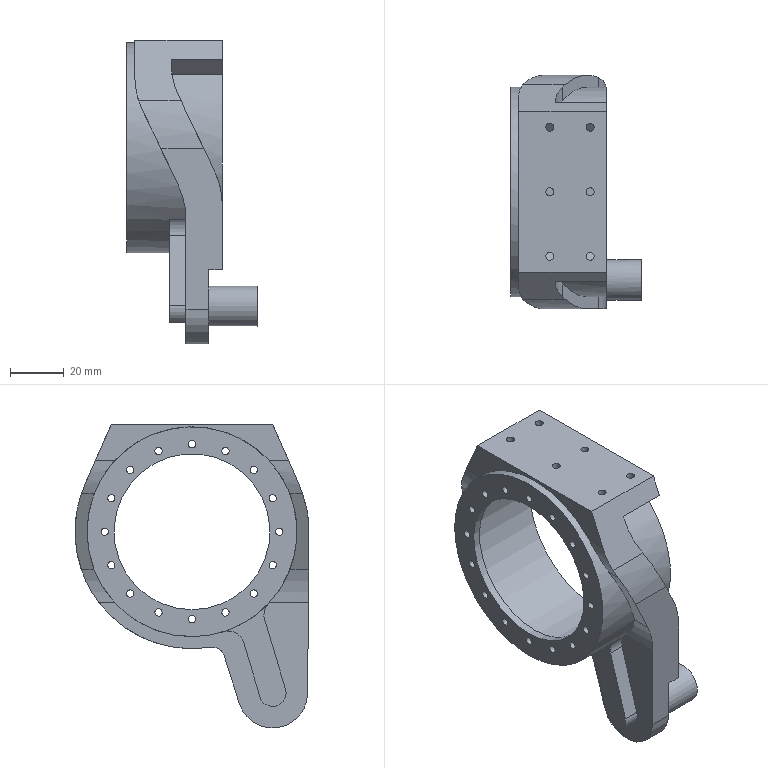Component | NX | TILT_BASE_ACC_1 | 1 solid | 74 faces | volume 76089 mm3 | cylinder 45 | plane 29 | commonest cylinder face diameters 2.7 x16 57 x8 3 x6 78 x3 87 x2 12 x2 70 x1 9 x1